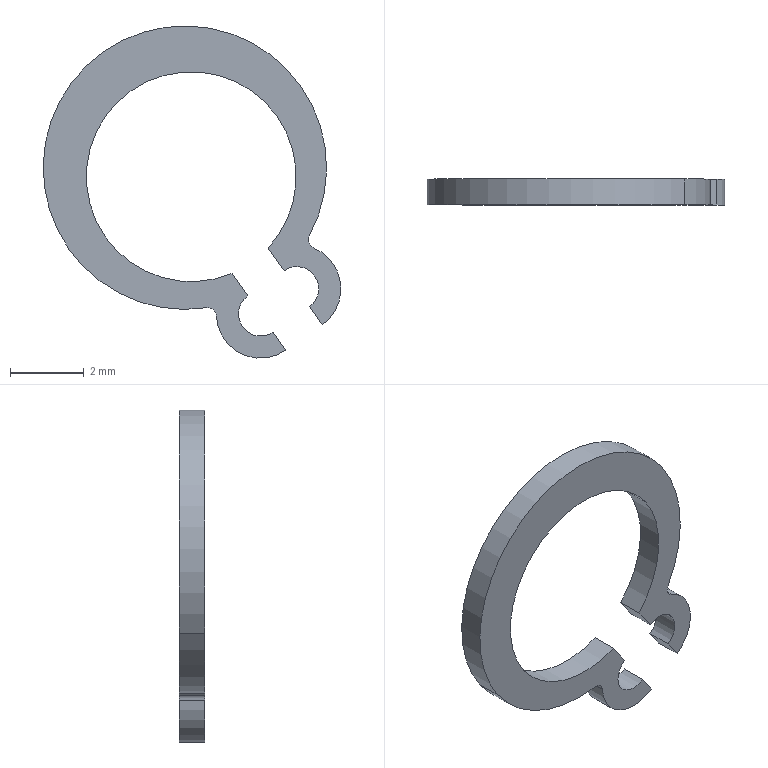Component | SolidWorks | JL001-03-06-1_GB_T894-2017[RetainingRingForShaftA-type(d0_9)6]-1 | 1 solid | 21 faces | box 8.09 x 0.7 x 9.03 mm | volume 16 mm3 | cylinder 15 | plane 6 | commonest cylinder face diameters 7.7 x3 0.48 x3 5.7 x3 1.2 x3 2.4 x3
build123d program:
from build123d import *

# Parameters (mm, degrees)
EXTRUDE1_DEPTH = 0.7


with BuildPart() as part:
    # Sketch → Extrude1 (new body)
    with BuildSketch(Plane.XY):
        with BuildLine():
            Line((-0.6, -2.786), (-0.6, -3.536))
            ThreePointArc((-0.6, -3.536), (-1.2, -4.136), (-0.6, -4.736))
            Line((-0.6, -4.736), (-0.6, -5.336))
            ThreePointArc((-0.6, -5.336), (-1.652, -4.714), (-1.613, -3.493))
            ThreePointArc((-1.613, -3.493), (-1.585, -3.3), (-1.709, -3.15))
            ThreePointArc((-1.709, -3.15), (0, 4.15), (1.709, -3.15))
            ThreePointArc((1.709, -3.15), (1.585, -3.3), (1.613, -3.493))
            ThreePointArc((1.613, -3.493), (1.652, -4.714), (0.6, -5.336))
            Line((0.6, -5.336), (0.6, -4.736))
            ThreePointArc((0.6, -4.736), (1.2, -4.136), (0.6, -3.536))
            Line((0.6, -3.536), (0.6, -2.786))
            ThreePointArc((0.6, -2.786), (0, 2.85), (-0.6, -2.786))
        make_face()
    extrude(amount=EXTRUDE1_DEPTH)


solid = part.part

# Placed as in the assembly
solid = solid.moved(Location((-69, 1039, 65), (90, 0, 35.038)))